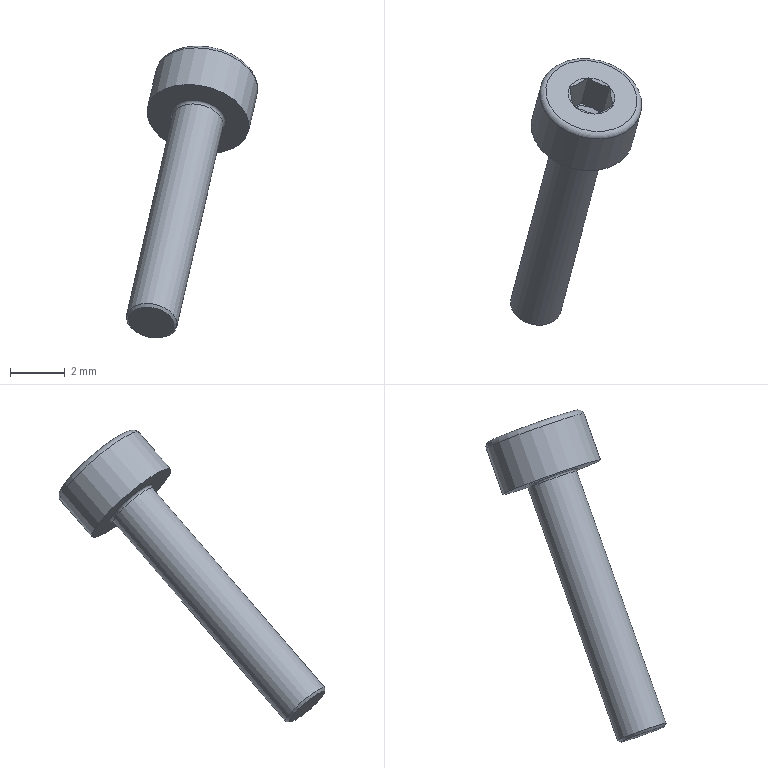Component | NX | GB-T70_1-2000_M2X10 | 1 solid | 27 faces | volume 47 mm3 | plane 15 | cone 8 | cylinder 2 | torus 2 | commonest cylinder face diameters 1.886 x1 3.8 x1